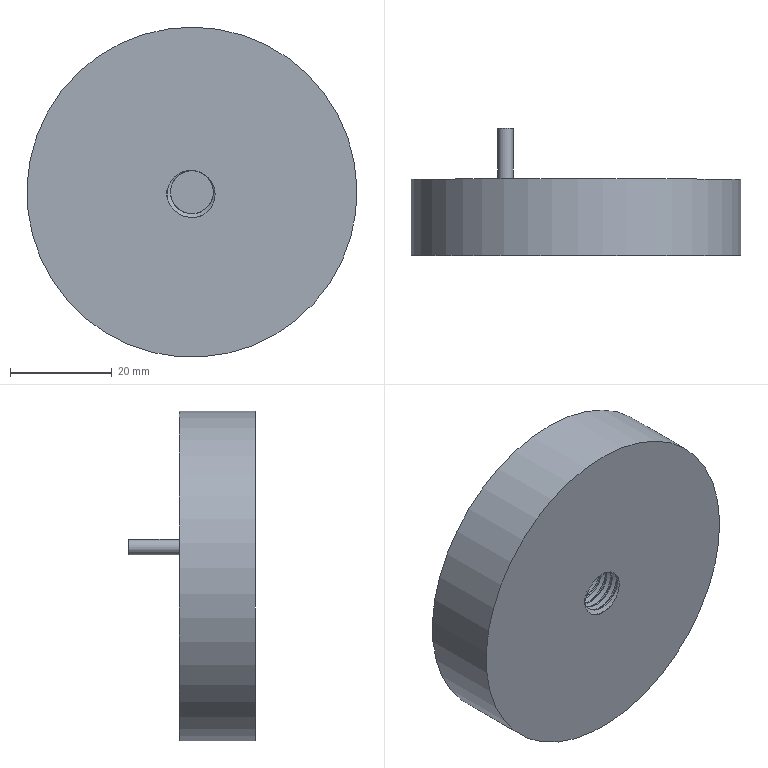Component | NX | MODEL1 | 1 solid | 14 faces | volume 46664 mm3 | plane 6 | cylinder 5 | spline 3 | commonest cylinder face diameters 8.5 x1 65 x1 40 x1 3 x1 10 x1